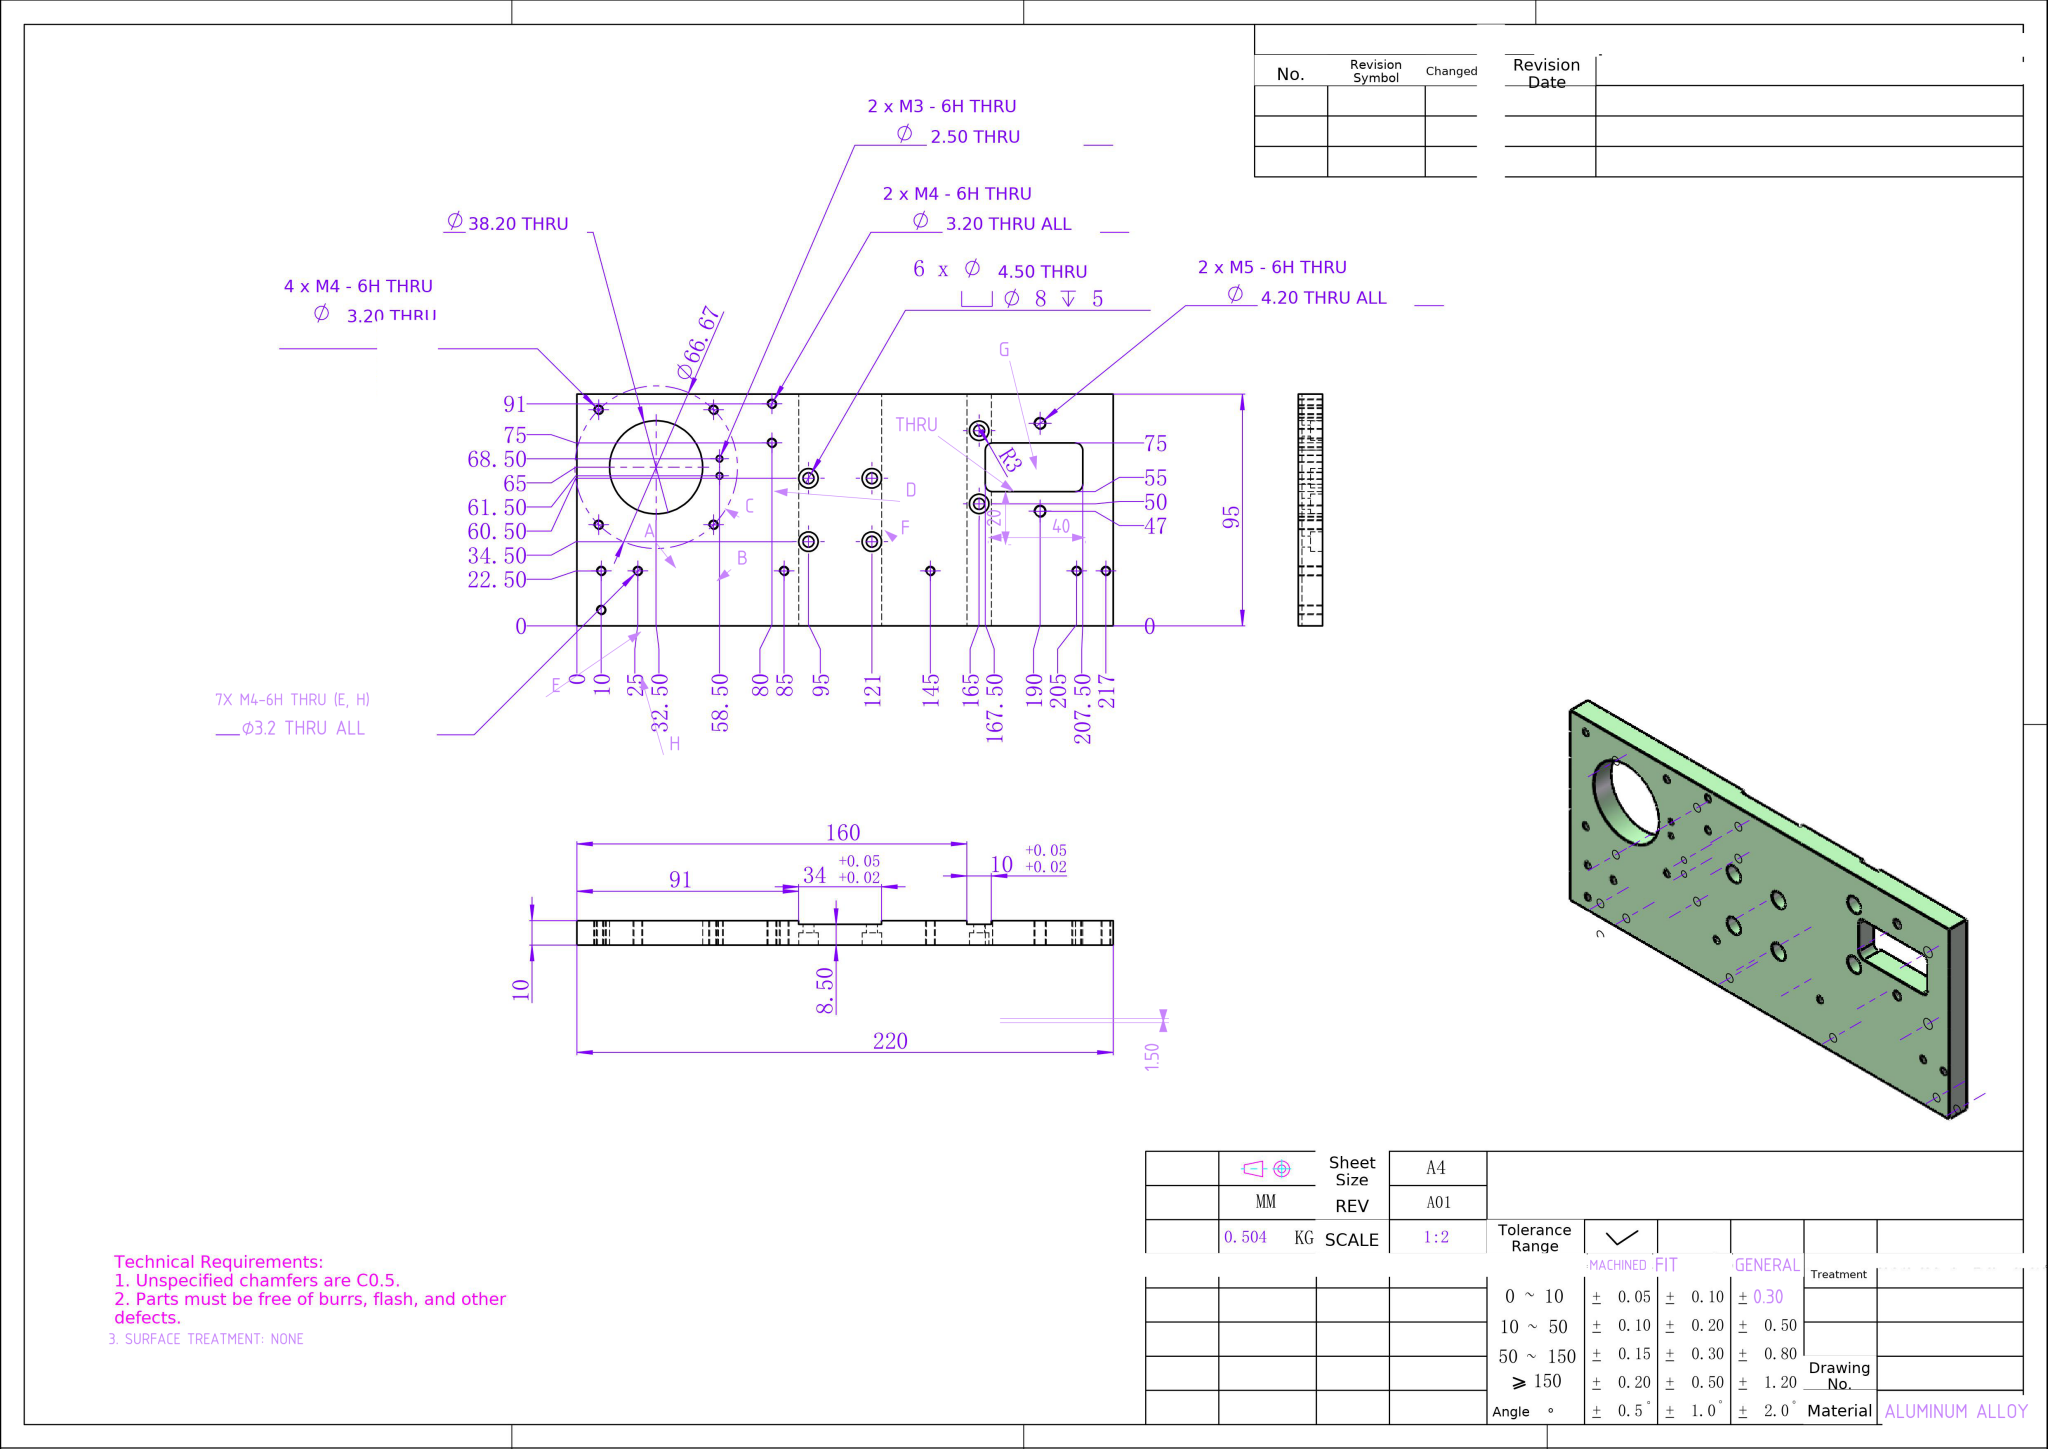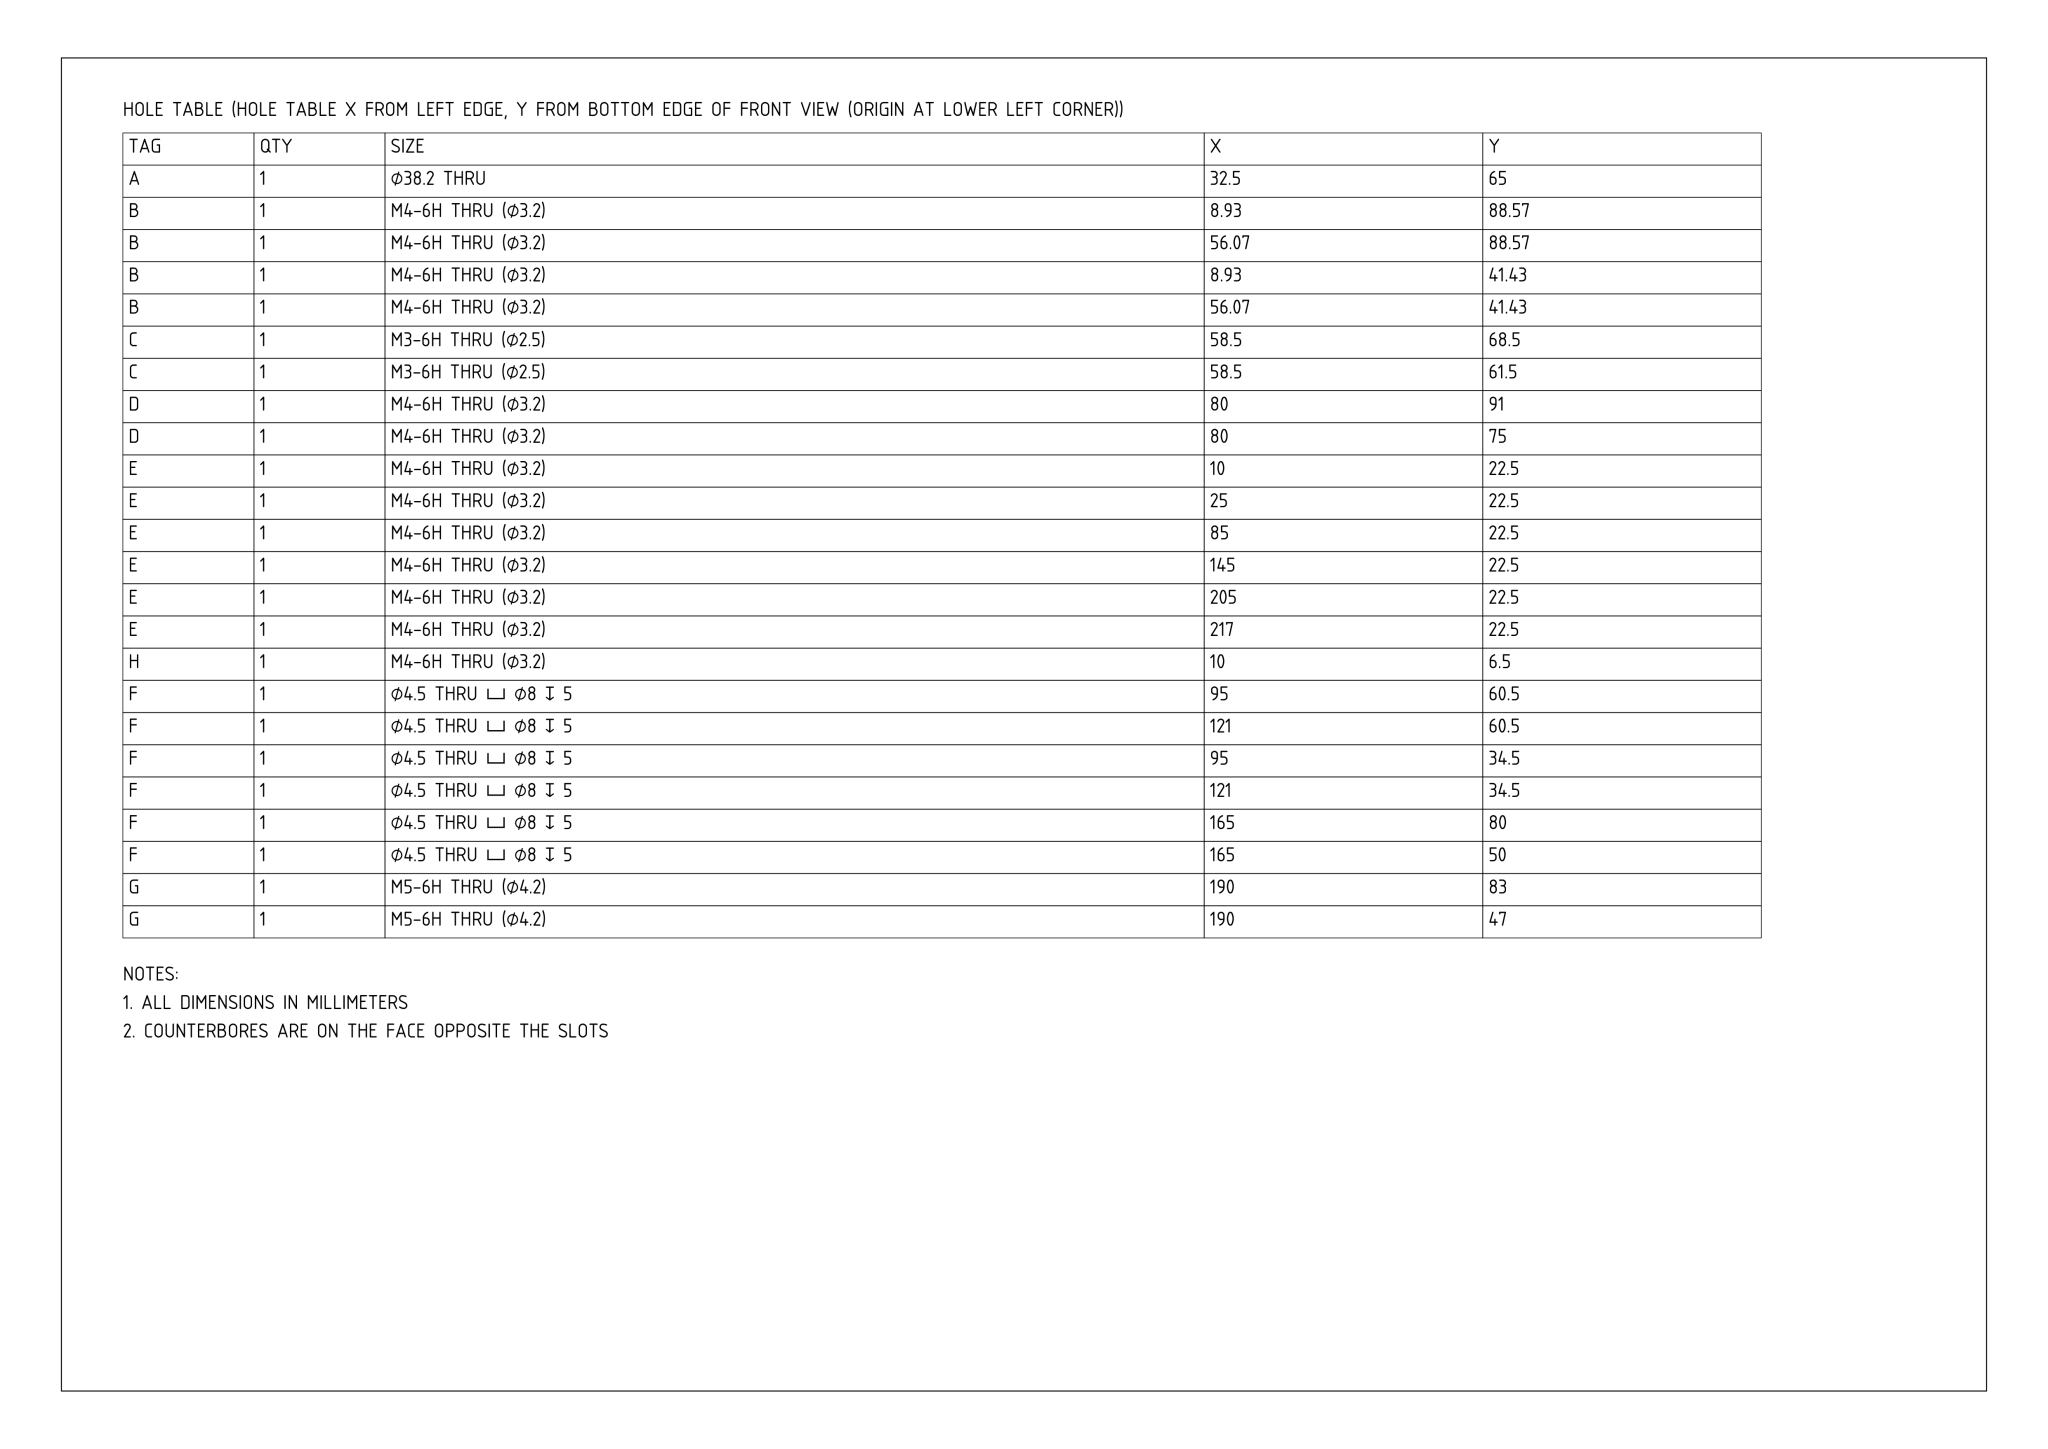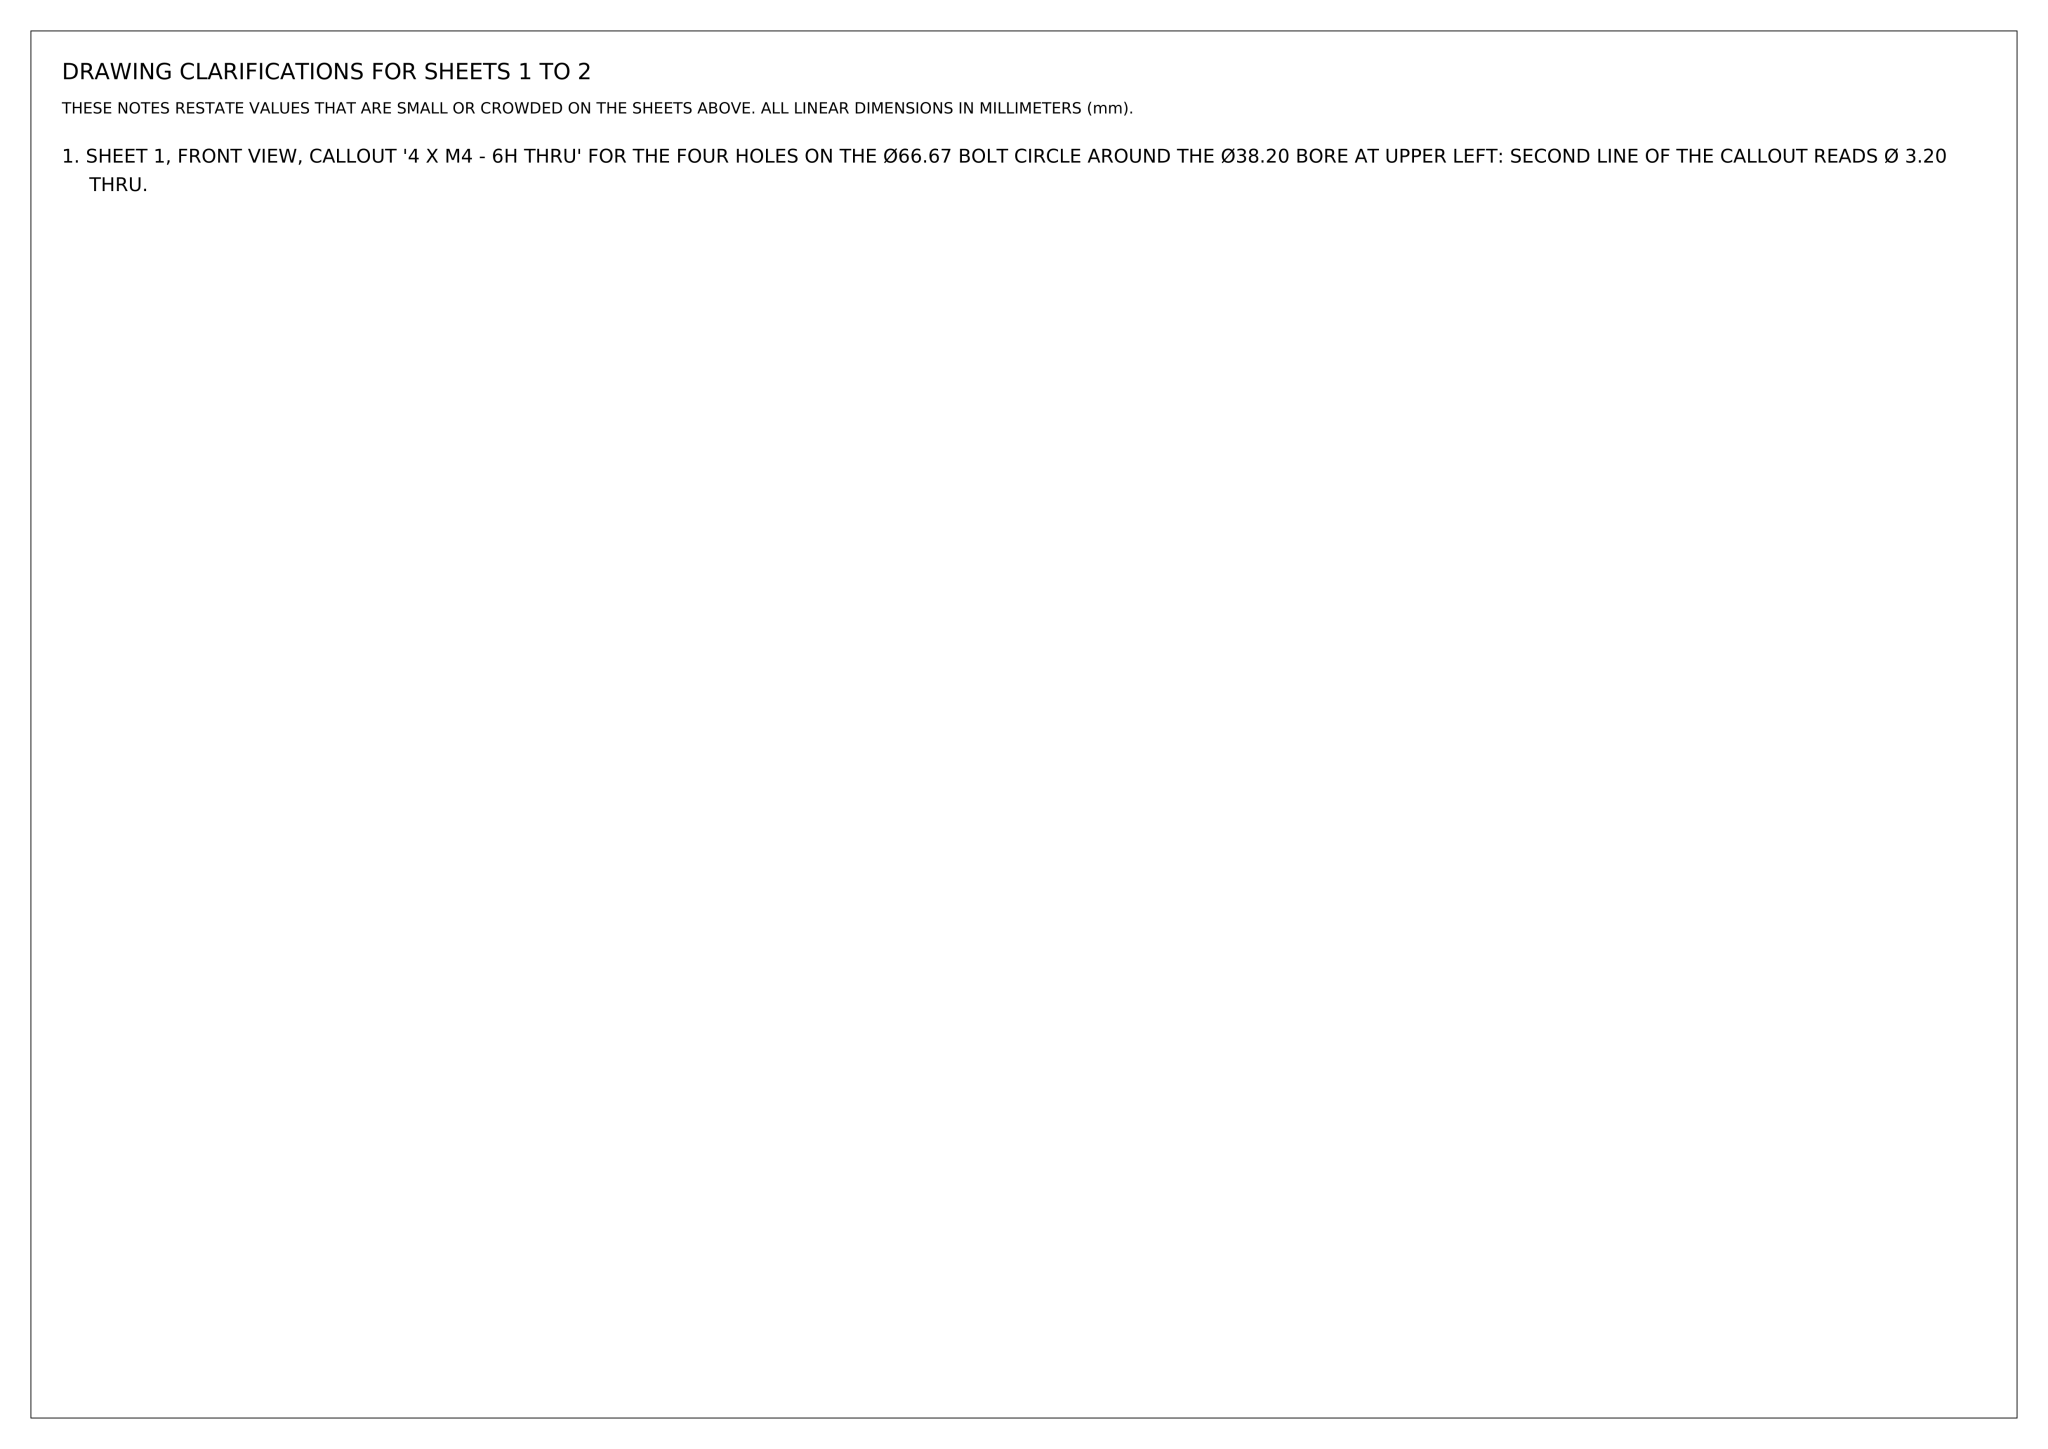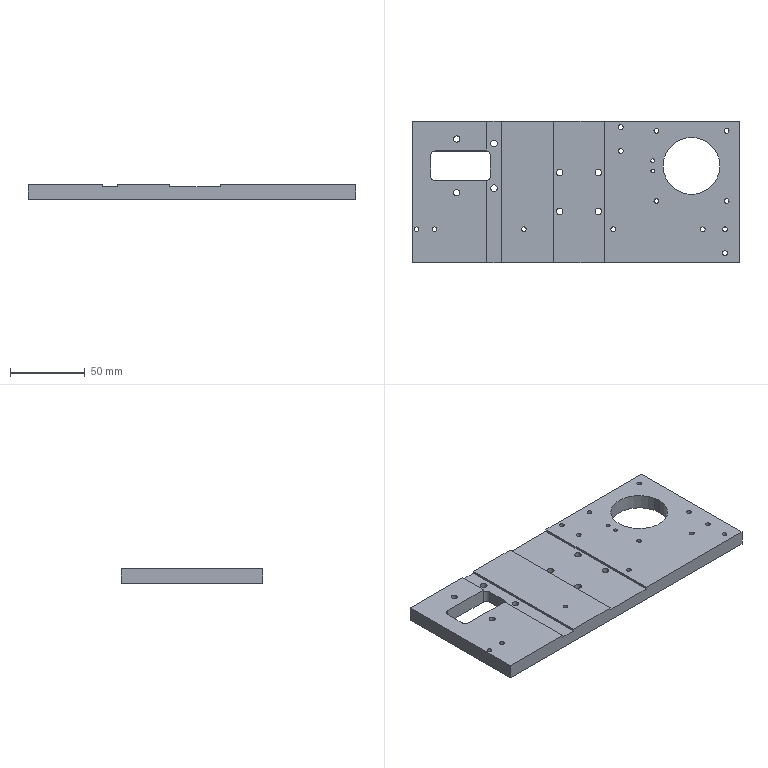Part | NX | mm | 1 solid | 89 faces | box 220 x 95 x 10 mm | volume 180153 mm3 | cylinder 64 | plane 25 | commonest cylinder face diameters 3.2 x26 8 x12 4.5 x12 4.2 x4 2.5 x4 6 x4 38.2 x2